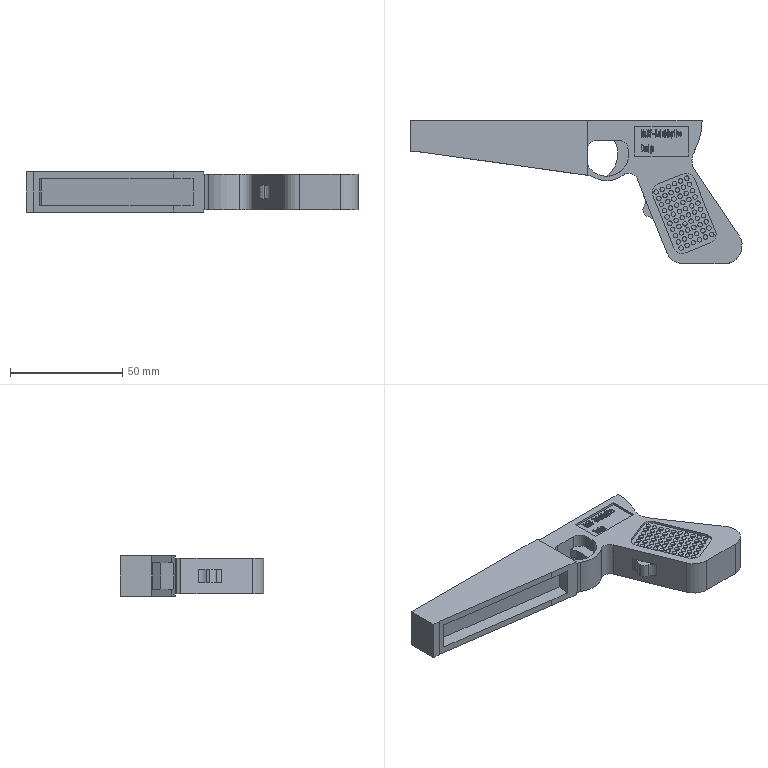Component | SolidWorks | Grip-1 | 1 solid | 946 faces | box 147.8 x 64 x 18 mm | volume 56001 mm3 | plane 440 | cylinder 273 | spline 233 | commonest cylinder face diameters 2 x240 8 x22 16 x4 6 x2 20 x1 24 x1 60 x1 3591.539 x1